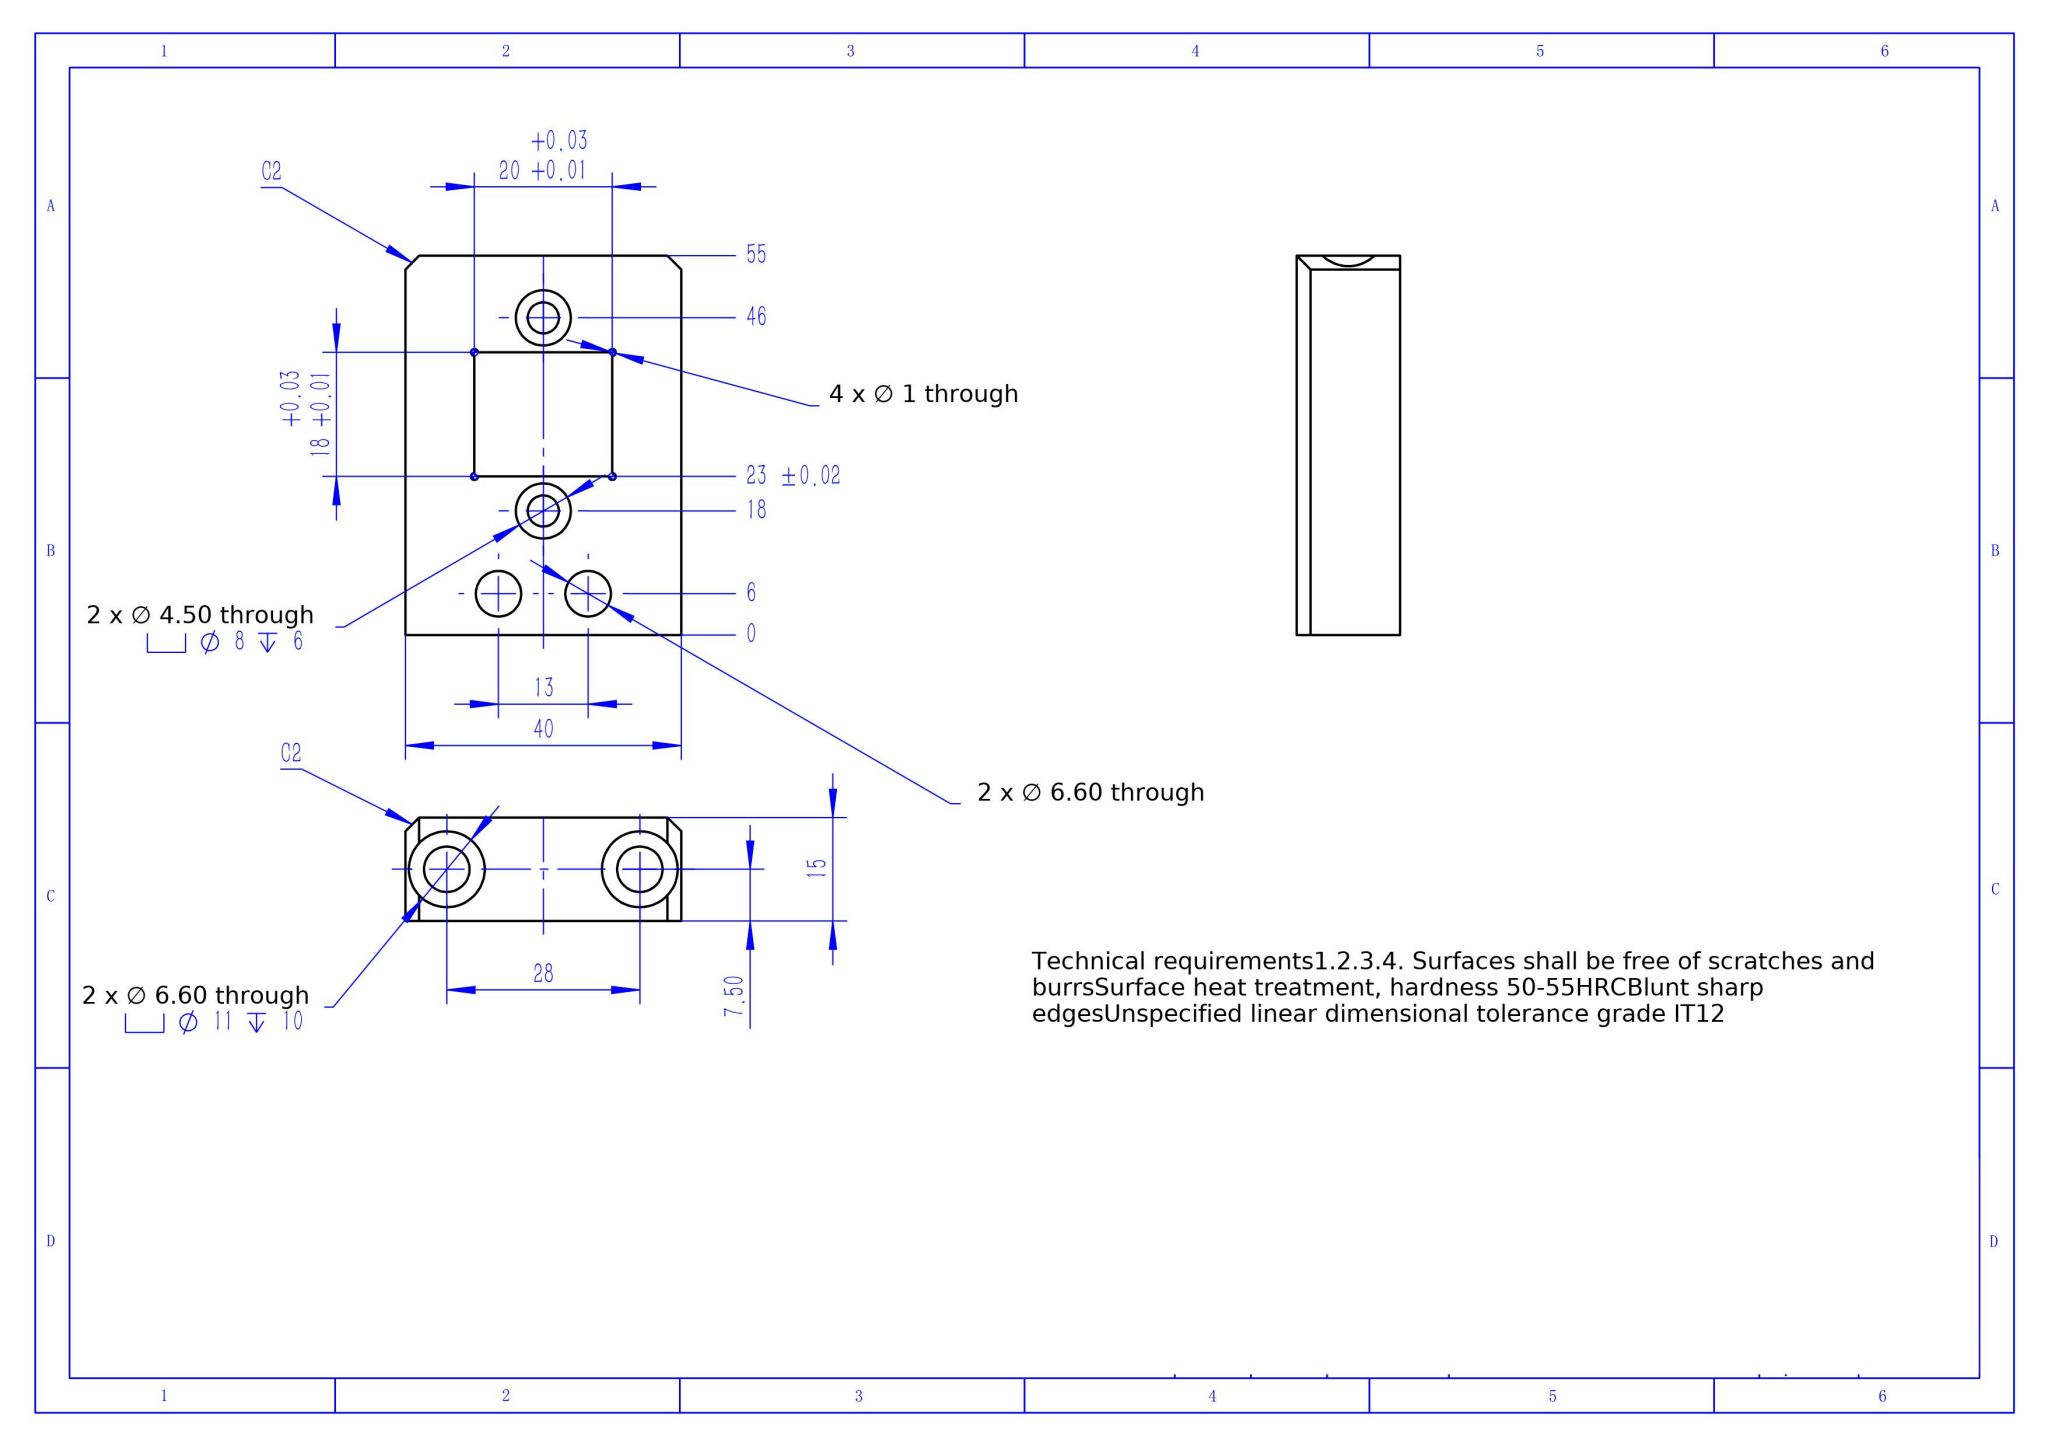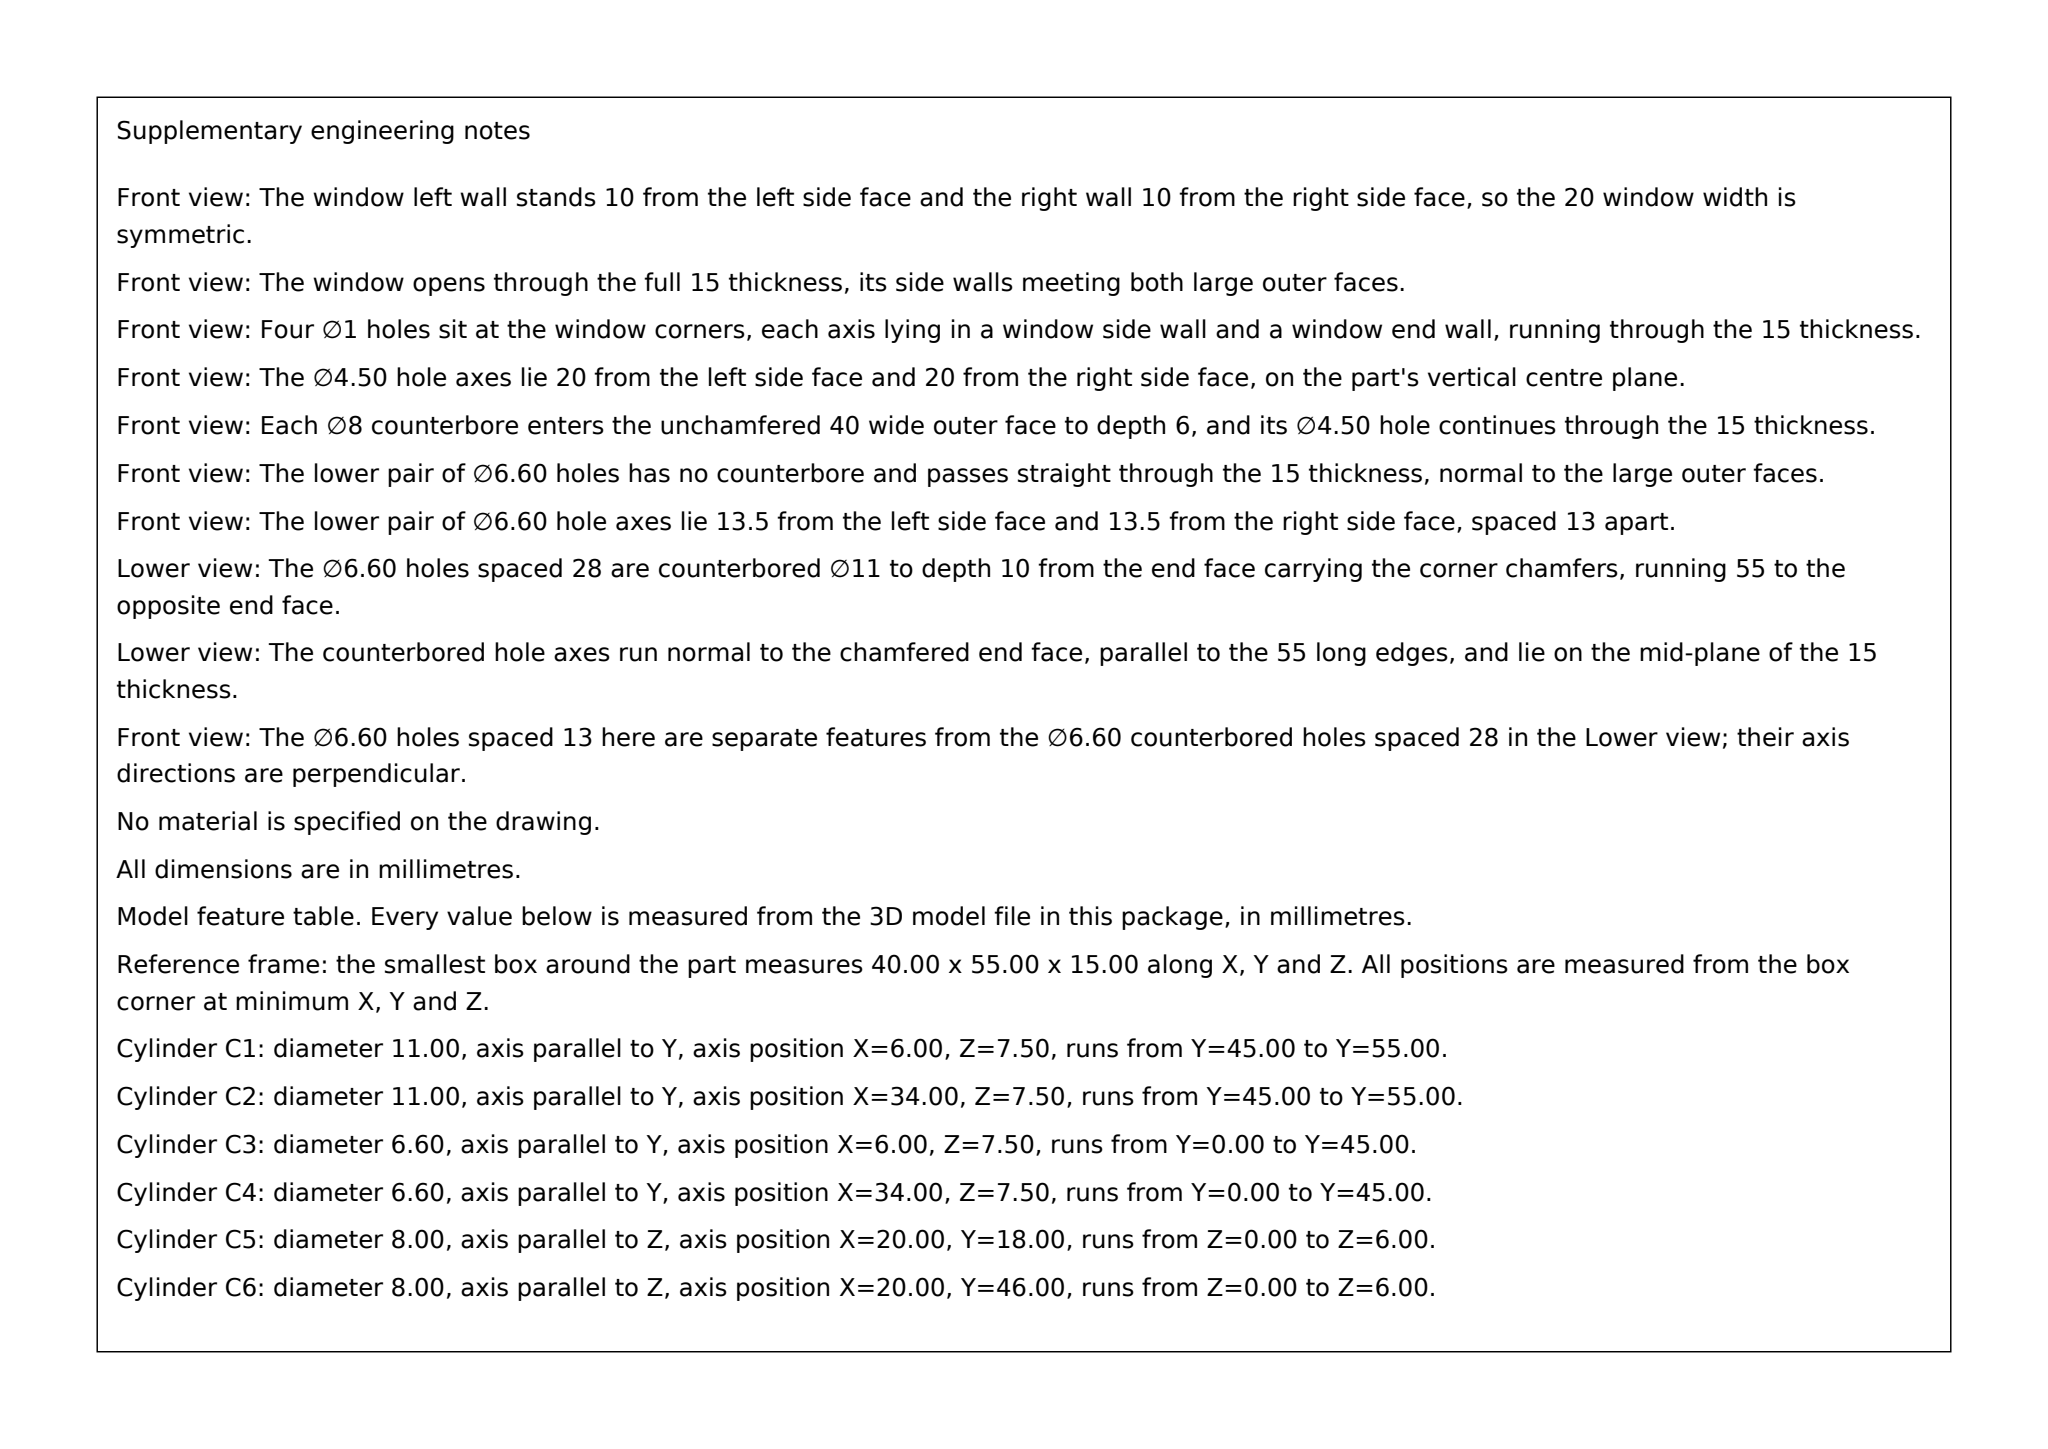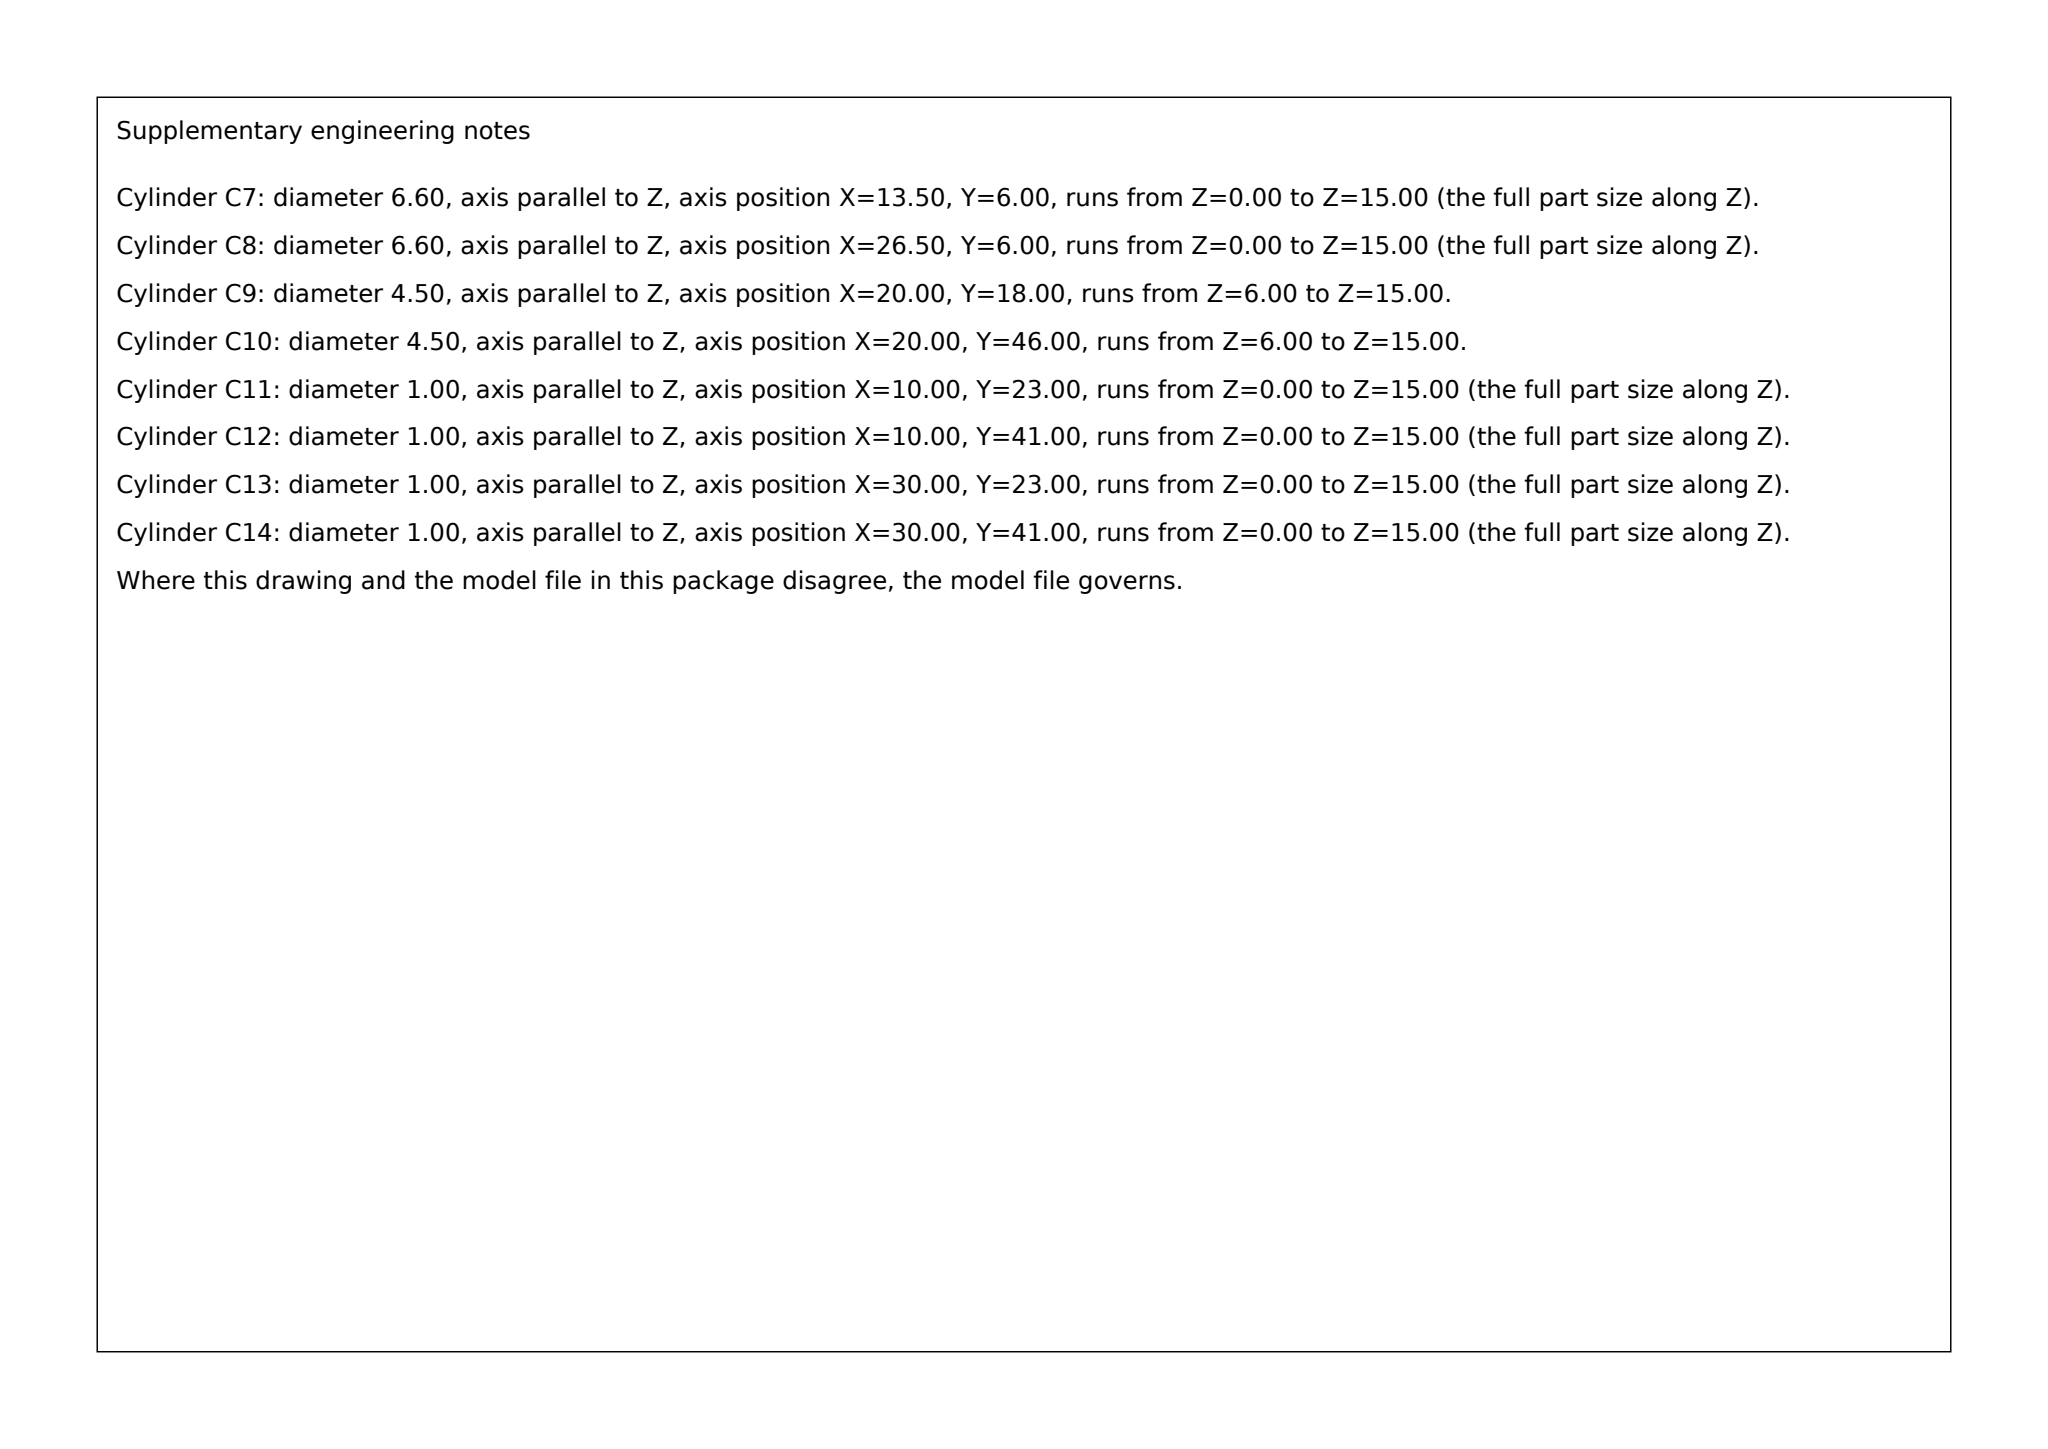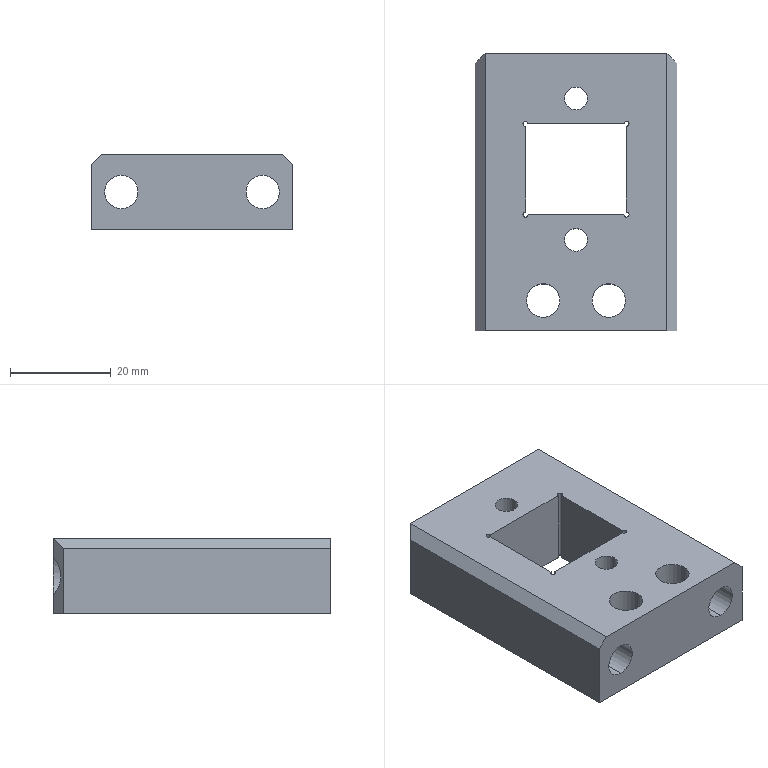Part | SolidWorks | mm | 1 solid | 44 faces | box 40 x 55 x 15 mm | volume 20404 mm3 | cylinder 26 | plane 18 | commonest cylinder face diameters 6.6 x8 1 x6 8 x4 4.5 x4 11 x4
Drawing notes:
2X Ø6.60 SIDE HOLES: DP 45 FROM Ø11 DP 10 C'BORE FLOOR, THRU 55 | from the solid: cylinders [6.6,'y',[6.0,null,7.5],45] & [6.6,'y',[34.0,null,7.5],45] with [11.0,'y',...,10]; y-planes at 45 (c'bore floors) and bbox Y=55